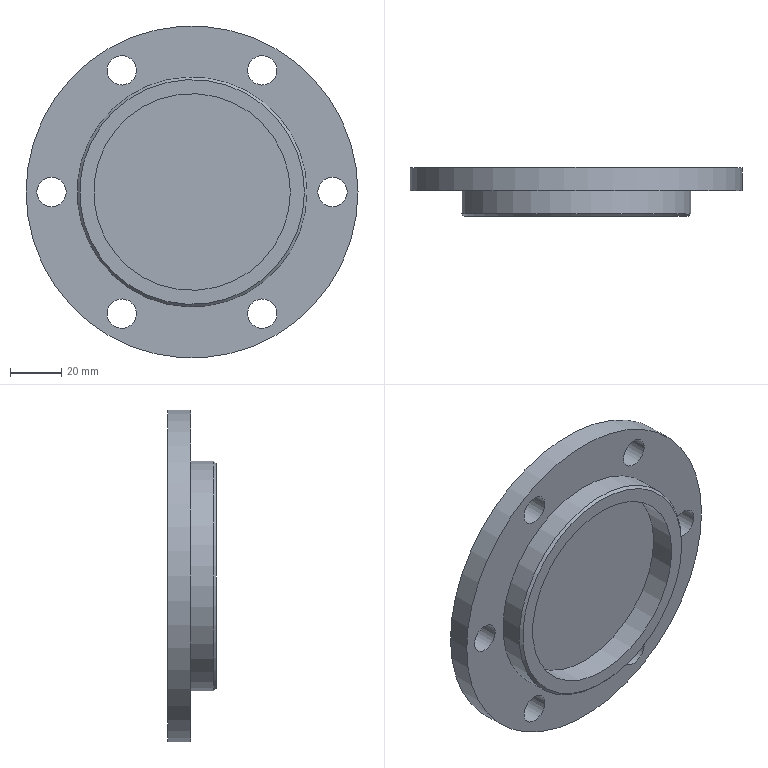Component | NX | END_CAP1 | 1 solid | 16 faces | volume 120708 mm3 | cylinder 10 | plane 5 | cone 1 | commonest cylinder face diameters 11.5 x6 130 x1 90 x1 77 x1 80 x1